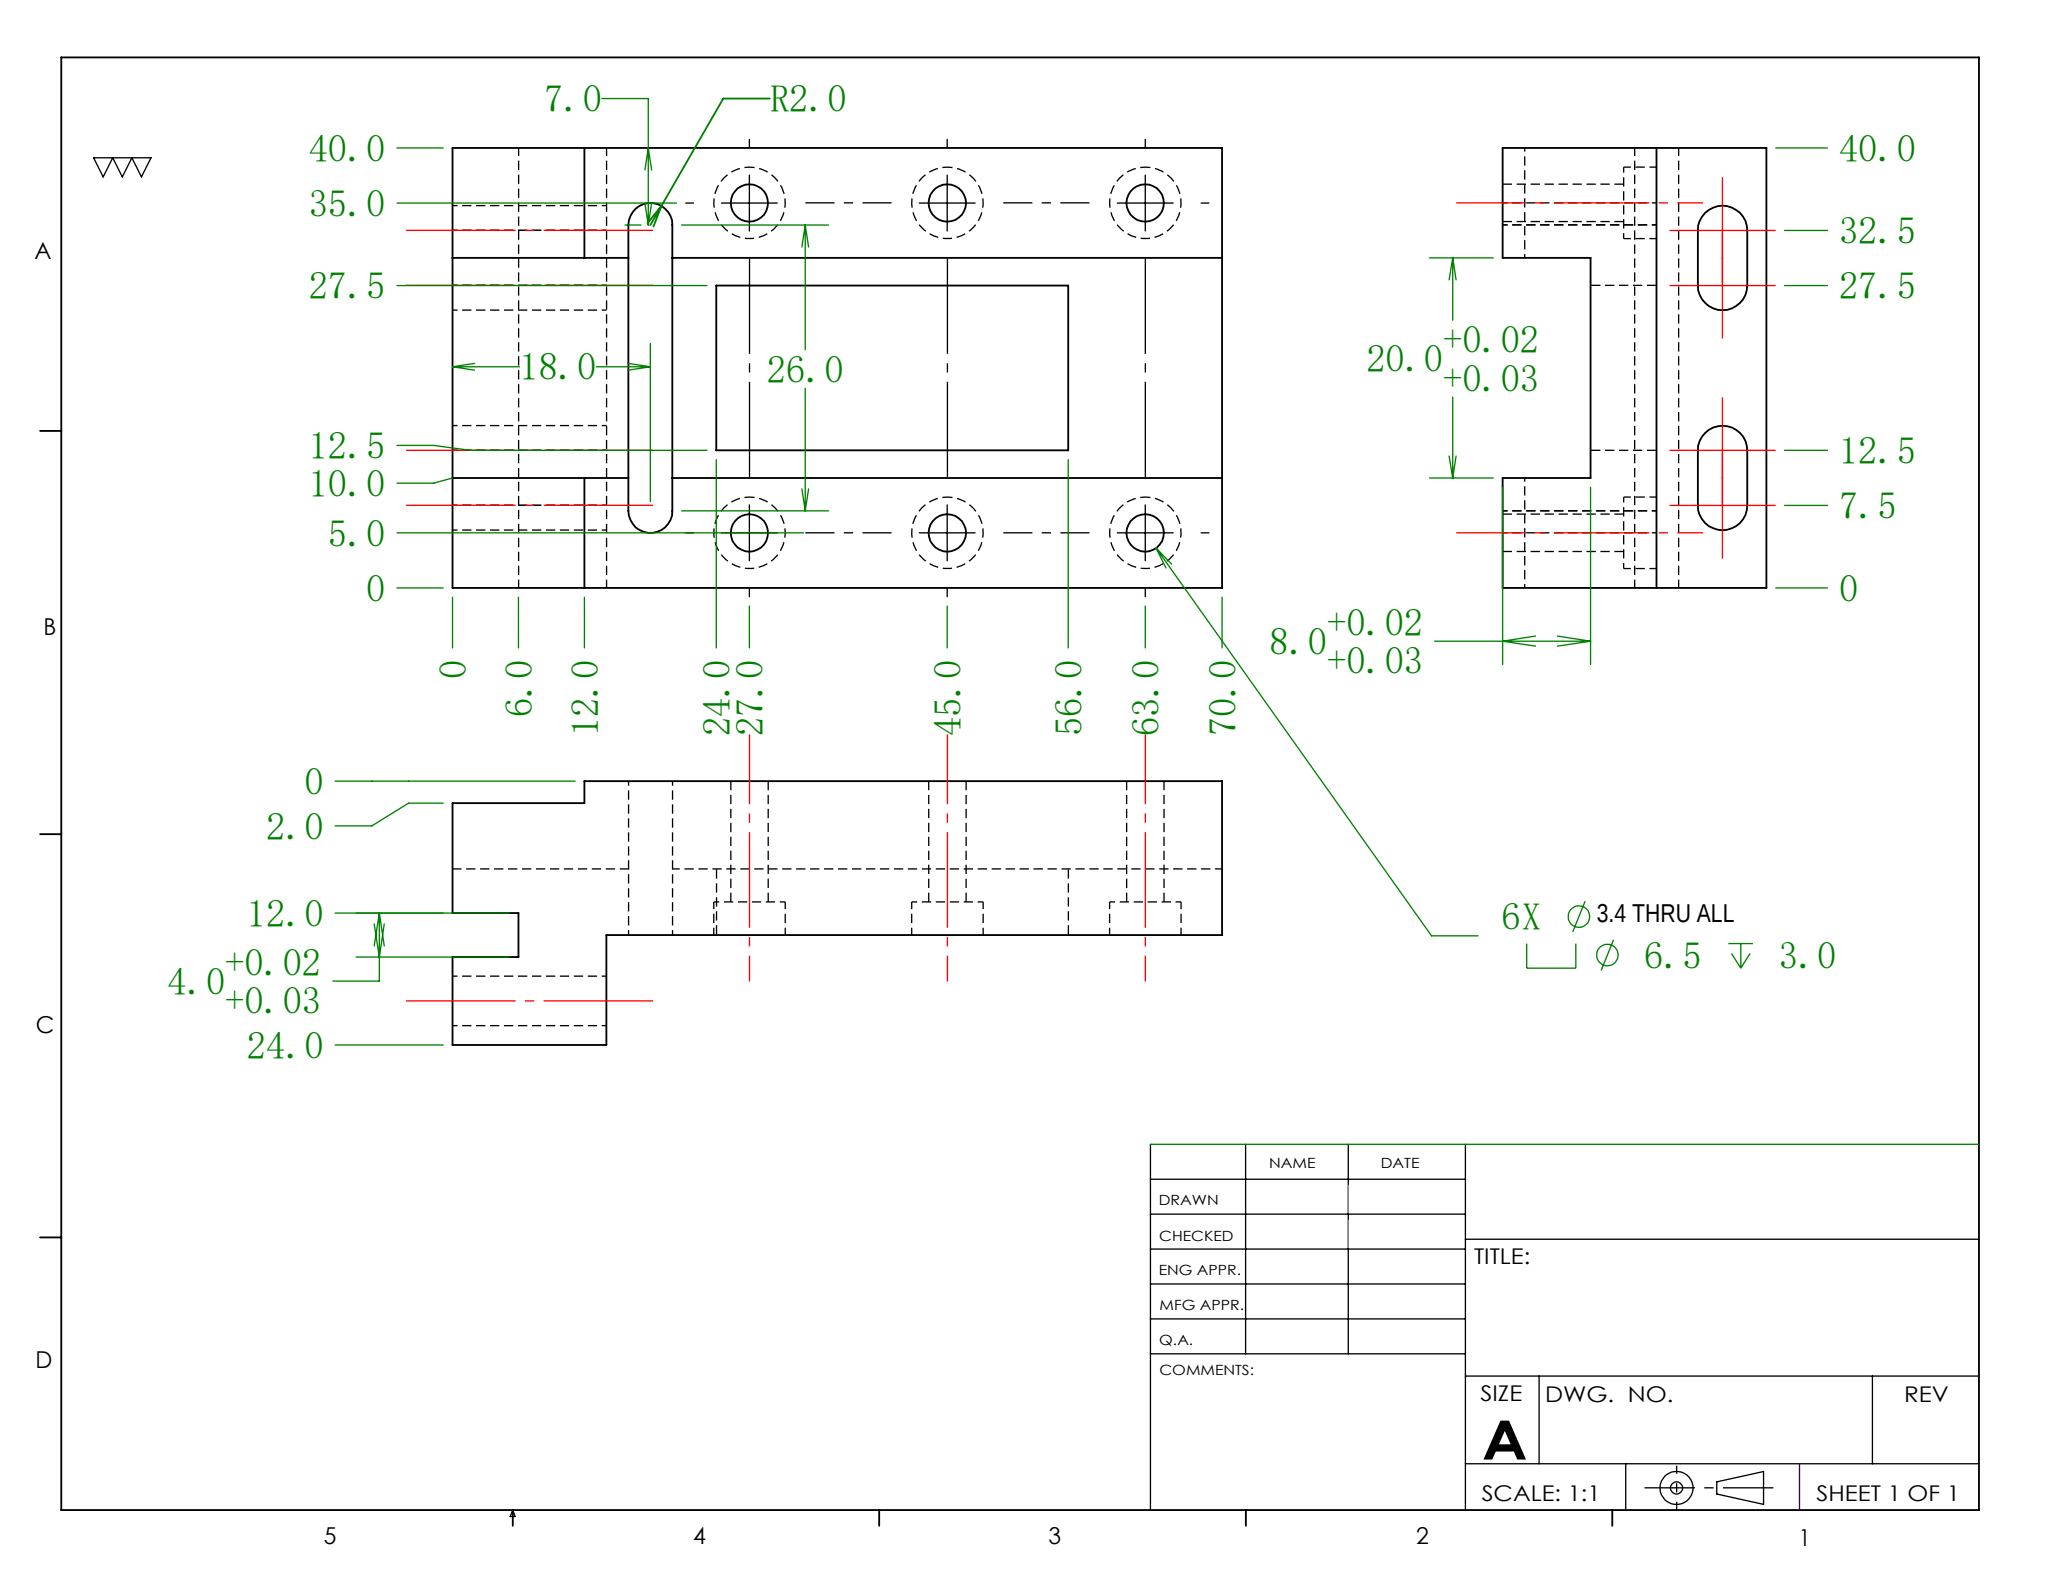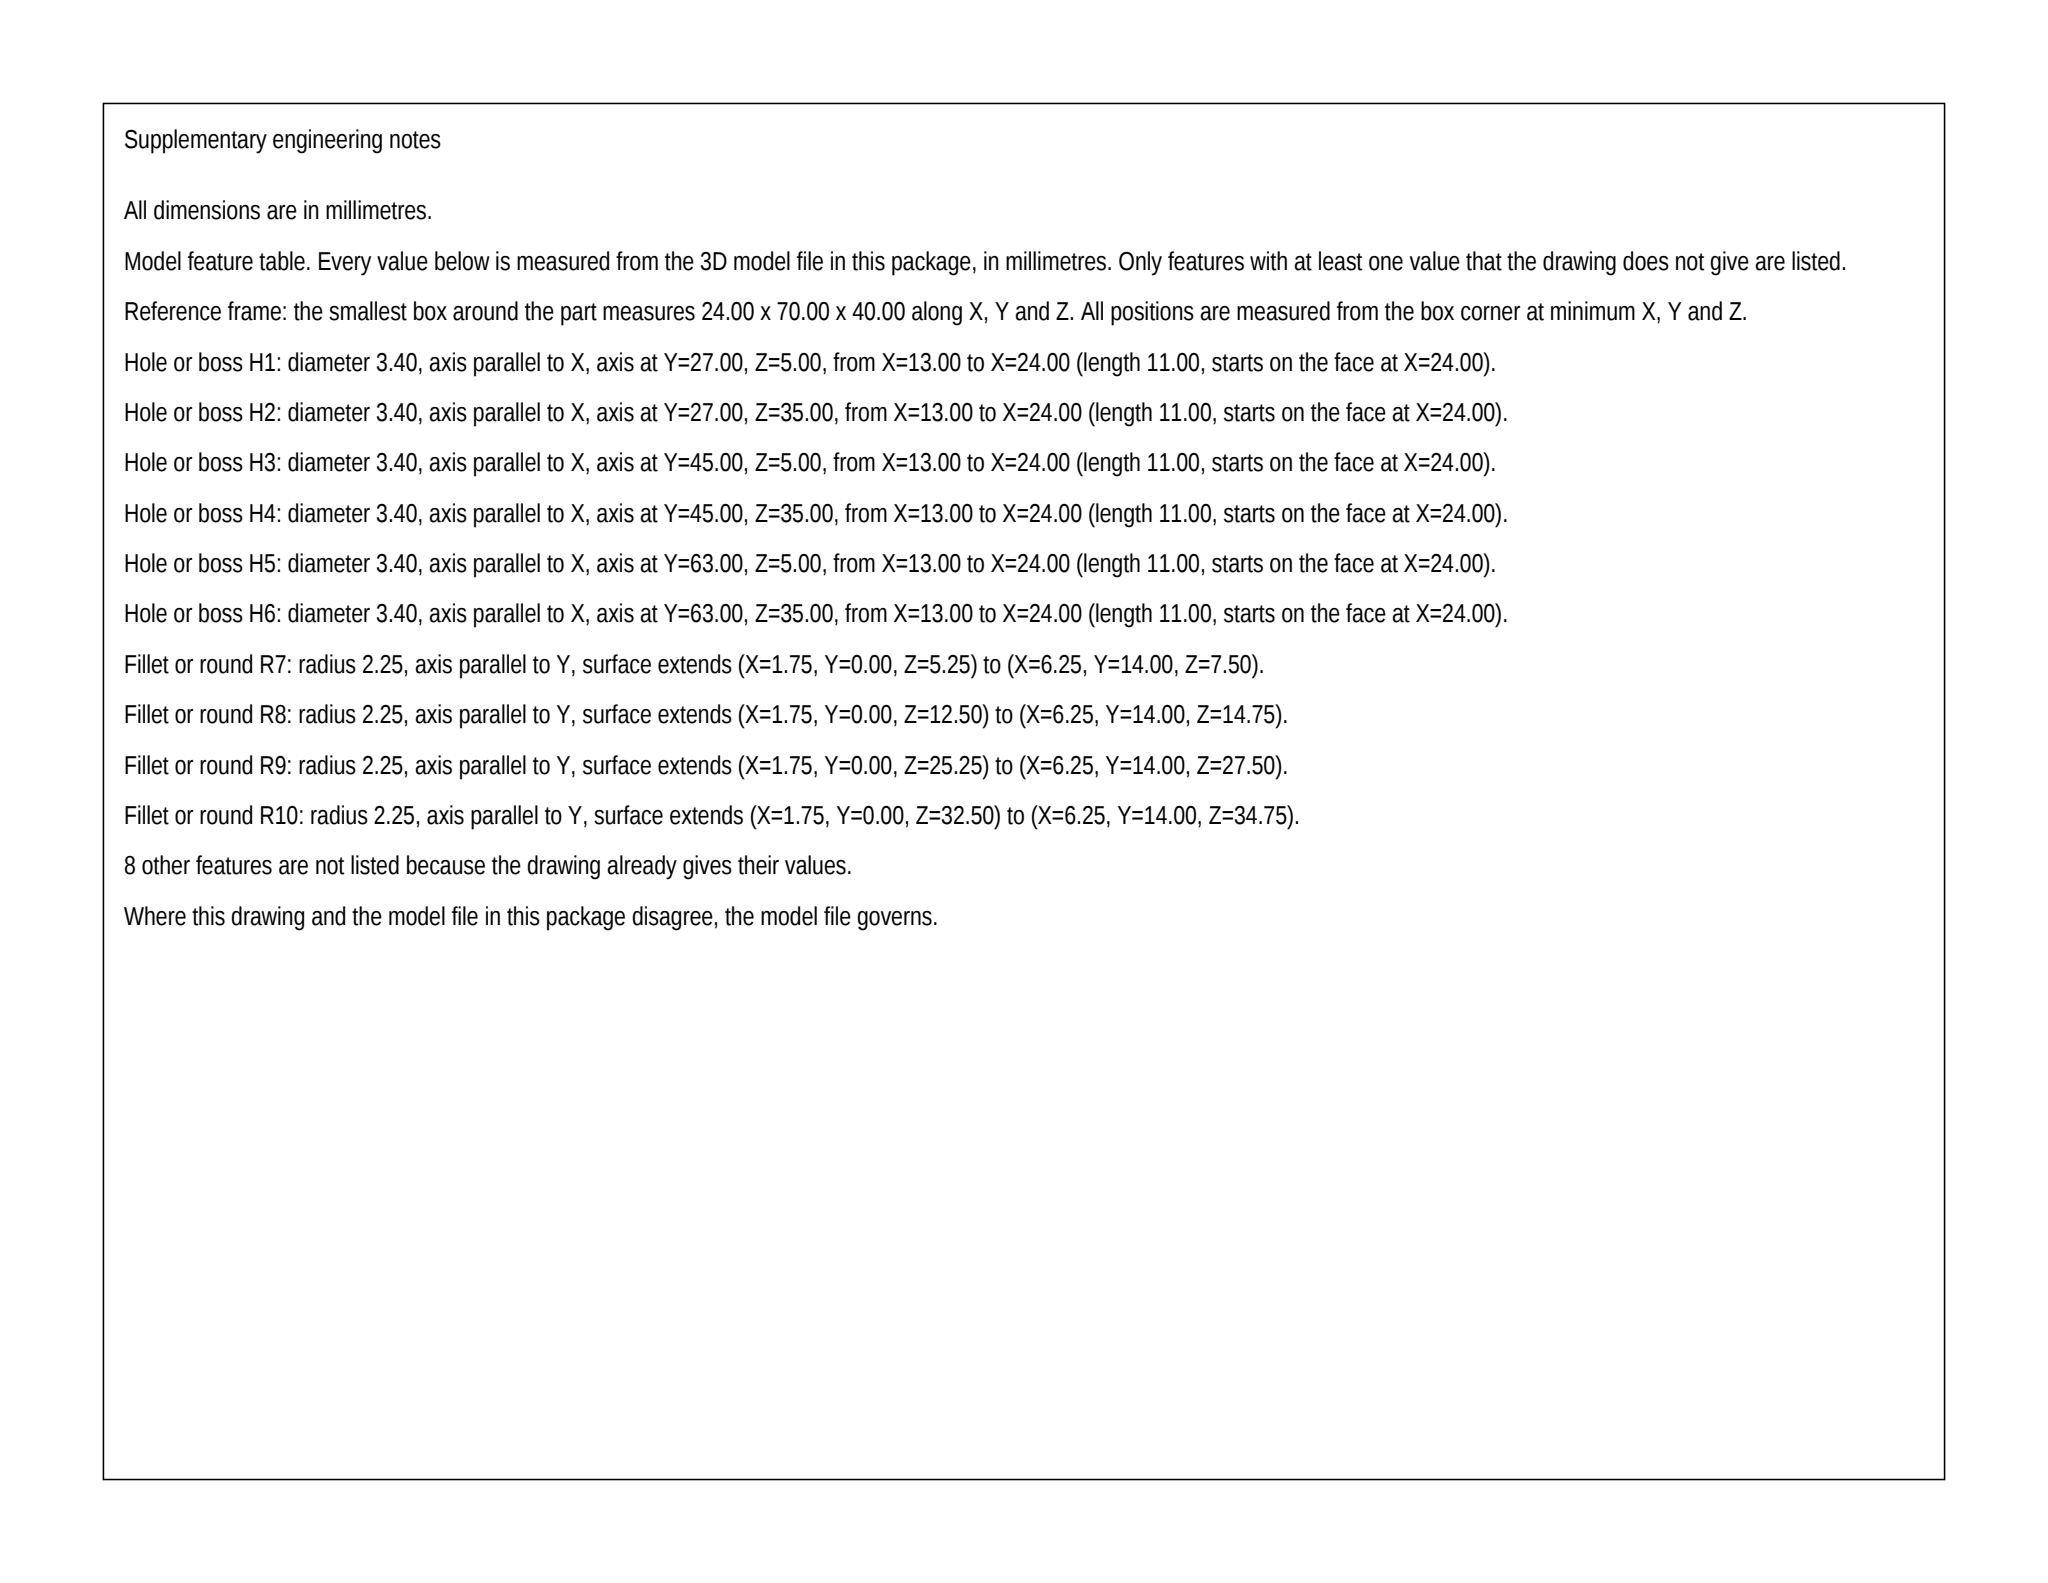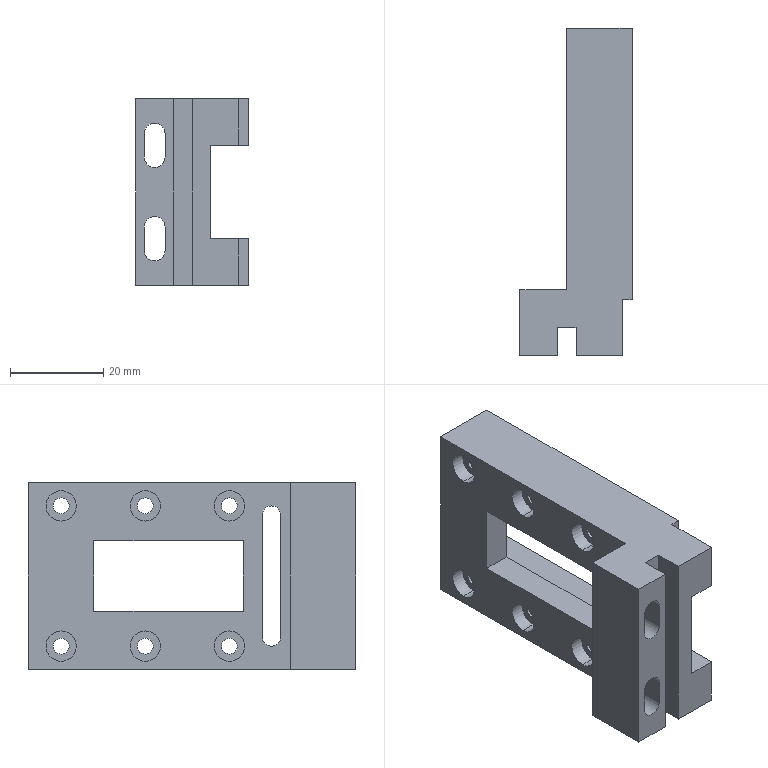Part | SolidWorks | mm | 1 solid | 72 faces | box 24 x 70 x 40 mm | volume 26016 mm3 | plane 39 | cylinder 33 | commonest cylinder face diameters 6.5 x12 3.4 x12 4.5 x6 4 x3
build123d program:
from build123d import *

# Parameters (mm, degrees)
SKETCH1_W                                            = 40
SKETCH1_H                                            = 70
EXTRUDE1_DEPTH                                       = 12
SKETCH2_W                                            = 20
SKETCH2_H                                            = 80
EXTRUDE2_DEPTH                                       = 8
SKETCH3_W                                            = 40
SKETCH3_H                                            = 14
EXTRUDE3_DEPTH                                       = 12
SKETCH4_W                                            = 4
SKETCH4_H                                            = 6
EXTRUDE4_DEPTH                                       = 82.511
EXTRUDE5_DEPTH                                       = 70.857
SKETCH12_W                                           = 40
SKETCH12_H                                           = 56
EXTRUDE6_DEPTH                                       = 2
CYLINDRICAL_COUNTERSUNK_HOLE_FOR_M3_SOCK_D           = 3.4
CYLINDRICAL_COUNTERSUNK_HOLE_FOR_M3_SOCK_CBORE_D     = 6.5
CYLINDRICAL_COUNTERSUNK_HOLE_FOR_M3_SOCK_CBORE_DEPTH = 3
LPATTERN1_COUNT                                      = 2
LPATTERN1_PITCH                                      = 30
LPATTERN1_COUNT_DIR2                                 = 3
LPATTERN1_PITCH_DIR2                                 = 18
SKETCH17_W                                           = 15
SKETCH17_H                                           = 28
EXTRUDE7_DEPTH                                       = 82.829
SKETCH18_W                                           = 6
SKETCH18_H                                           = 15
EXTRUDE8_DEPTH                                       = 4
SKETCH19_W                                           = 40
SKETCH19_H                                           = 12
EXTRUDE9_DEPTH                                       = 2
CUT_EXTRUDE1_DEPTH                                   = 82.829


with BuildPart() as part:
    # Sketch1 → Extrude1 (new body)
    with BuildSketch(Plane(origin=(0, 0, 0), x_dir=(0, 0, -1), z_dir=(1, 0, 0))):
        with Locations((20, 35)):
            Rectangle(SKETCH1_W, SKETCH1_H)
    extrude(amount=EXTRUDE1_DEPTH)

    # Sketch2 → Extrude2 (cut)
    with BuildSketch(Plane(origin=(12, 0, 0), x_dir=(0, 0, -1), z_dir=(1, 0, 0))):
        with Locations((20, 30)):
            Rectangle(SKETCH2_W, SKETCH2_H)
    extrude(amount=-EXTRUDE2_DEPTH, mode=Mode.SUBTRACT)

    # Sketch3 → Extrude3 (add)
    with BuildSketch(Plane.ZY):
        with Locations((-20, 7)):
            Rectangle(SKETCH3_W, SKETCH3_H)
    extrude(amount=EXTRUDE3_DEPTH)

    # Sketch4 → Extrude4 (cut, through all)
    with BuildSketch(Plane(origin=(0, 0, -40), x_dir=(-1, 0, 0), z_dir=(0, 0, -1))):
        with Locations((2, 3)):
            Rectangle(SKETCH4_W, SKETCH4_H)
    extrude(amount=-EXTRUDE4_DEPTH, mode=Mode.SUBTRACT)

    # Sketch5 → Extrude5 (cut, through all)
    with BuildSketch(Plane(origin=(0, 14, 0), x_dir=(1, 0, 0), z_dir=(0, 1, 0))):
        with BuildLine():
            Line((-5.75, 32.5), (-5.75, 27.5))
            ThreePointArc((-5.75, 27.5), (-8, 25.25), (-10.25, 27.5))
            Line((-10.25, 27.5), (-10.25, 32.5))
            ThreePointArc((-10.25, 32.5), (-8, 34.75), (-5.75, 32.5))
        make_face()
        with BuildLine():
            Line((-5.75, 12.5), (-5.75, 7.5))
            ThreePointArc((-5.75, 7.5), (-8, 5.25), (-10.25, 7.5))
            Line((-10.25, 7.5), (-10.25, 12.5))
            ThreePointArc((-10.25, 12.5), (-8, 14.75), (-5.75, 12.5))
        make_face()
    extrude(amount=-EXTRUDE5_DEPTH, mode=Mode.SUBTRACT)

    # Sketch12 → Extrude6 (add)
    with BuildSketch(Plane.ZY):
        with Locations((-20, 42)):
            Rectangle(SKETCH12_W, SKETCH12_H)
    extrude(amount=EXTRUDE6_DEPTH)

    # Cylindrical Countersunk Hole for M3 Sock (through all)
    with Locations(Plane.ZY.offset(2)):
        with Locations((-35, 63)):
            cylindrical_countersunk_hole_for_m3_sock = CounterBoreHole(CYLINDRICAL_COUNTERSUNK_HOLE_FOR_M3_SOCK_D / 2, CYLINDRICAL_COUNTERSUNK_HOLE_FOR_M3_SOCK_CBORE_D / 2, CYLINDRICAL_COUNTERSUNK_HOLE_FOR_M3_SOCK_CBORE_DEPTH)

    # LPattern1: Cylindrical Countersunk Hole for M3 Sock 2 × 3
    with Locations(*[(0, -j * LPATTERN1_PITCH_DIR2, i * LPATTERN1_PITCH) for i in range(LPATTERN1_COUNT) for j in range(LPATTERN1_COUNT_DIR2) if (i, j) != (0, 0)]):
        add(cylindrical_countersunk_hole_for_m3_sock, mode=Mode.SUBTRACT)

    # Sketch17 → Extrude7 (cut, through all)
    with BuildSketch(Plane.ZY.offset(2)):
        with Locations((-20, 42)):
            Rectangle(SKETCH17_W, SKETCH17_H)
    extrude(amount=-EXTRUDE7_DEPTH, mode=Mode.SUBTRACT)

    # Sketch18 → Extrude8 (cut)
    with BuildSketch(Plane(origin=(0, 28, 0), x_dir=(1, 0, 0), z_dir=(0, 1, 0))):
        with Locations((1, 20)):
            Rectangle(SKETCH18_W, SKETCH18_H)
    extrude(amount=-EXTRUDE8_DEPTH, mode=Mode.SUBTRACT)

    # Sketch19 → Extrude9 (cut)
    with BuildSketch(Plane(origin=(12, 0, 0), x_dir=(0, 0, -1), z_dir=(1, 0, 0))):
        with Locations((20, 6)):
            Rectangle(SKETCH19_W, SKETCH19_H)
    extrude(amount=-EXTRUDE9_DEPTH, mode=Mode.SUBTRACT)

    # Sketch20 → Cut-Extrude1 (cut, through all)
    with BuildSketch(Plane.ZY.offset(2)):
        with BuildLine():
            Line((-33, 20), (-7, 20))
            ThreePointArc((-7, 20), (-5, 18), (-7, 16))
            Line((-7, 16), (-33, 16))
            ThreePointArc((-33, 16), (-35, 18), (-33, 20))
        make_face()
    extrude(amount=-CUT_EXTRUDE1_DEPTH, mode=Mode.SUBTRACT)


solid = part.part